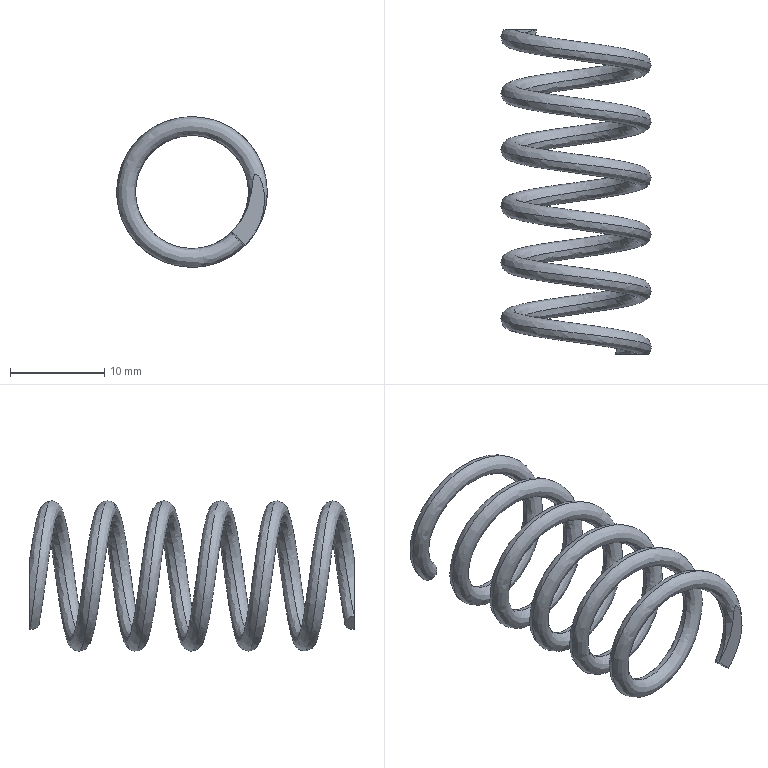Component | SolidWorks | CylindricalHelicalCompressionSpring-2 | 1 solid | 6 faces | volume 792 mm3 | plane 4 | spline 2